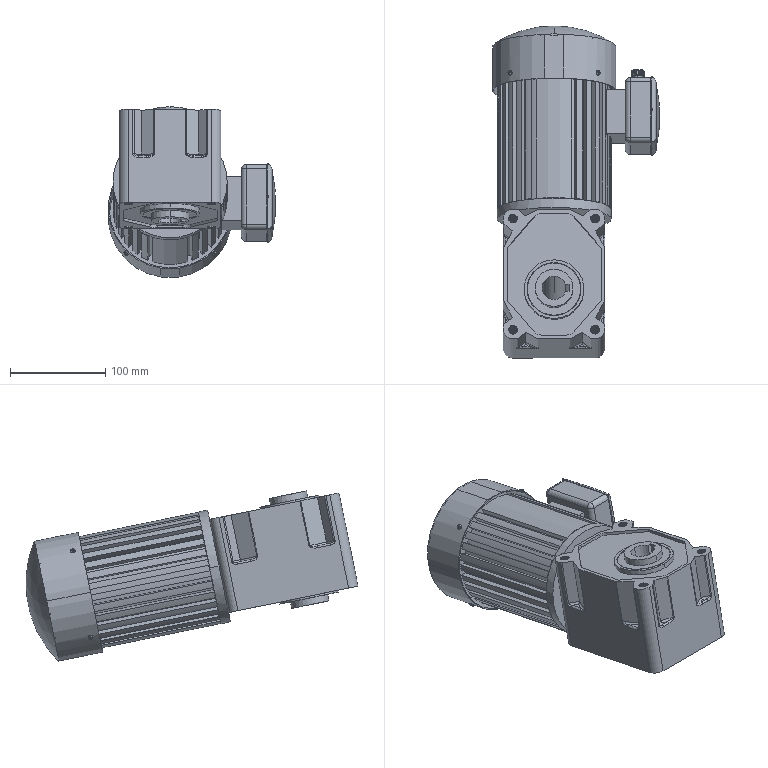Component | SolidWorks | HGF2_S400M-1 | 2 solids | 744 faces | volume 3193128 mm3 | plane 364 | cylinder 327 | spline 29 | torus 16 | sphere 6 | cone 2 | commonest cylinder face diameters 8.5 x168 4 x40 120 x38 5 x16 13 x15 20 x12 10 x8 56 x4